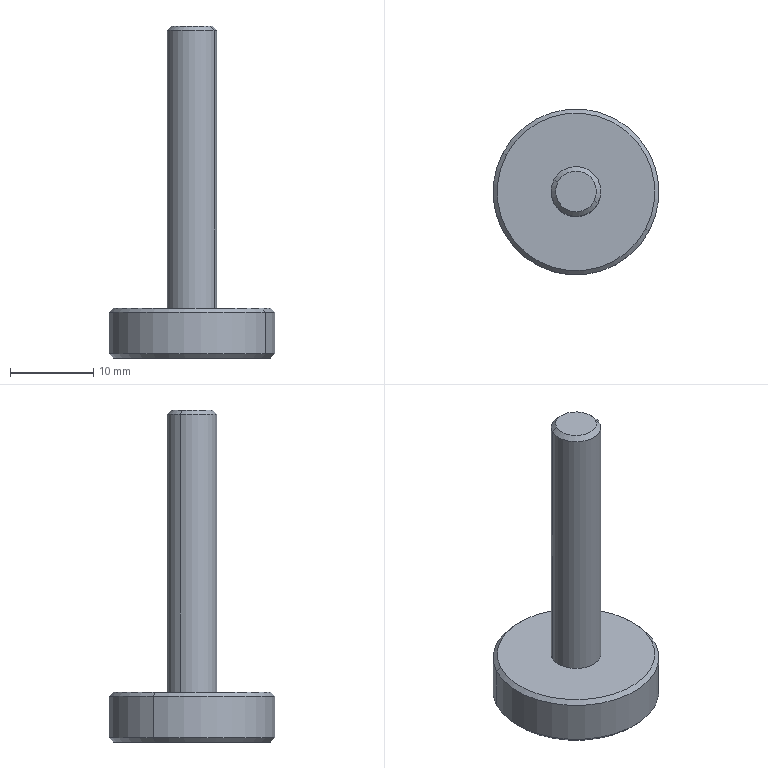Component | SolidWorks | 33KnurledScrew-1 | 1 solid | 13 faces | box 20 x 20 x 40 mm | volume 2828 mm3 | cone 6 | cylinder 4 | plane 3 | commonest cylinder face diameters 6 x2 20 x2
STEP:
#1=COLOUR_RGB('',0.7922,0.8196,0.9333);
#2=FILL_AREA_STYLE_COLOUR('',#1);
#3=FILL_AREA_STYLE('',(#2));
#4=SURFACE_STYLE_FILL_AREA(#3);
#5=SURFACE_SIDE_STYLE('',(#4));
#6=SURFACE_STYLE_USAGE(.BOTH.,#5);
#7=PRESENTATION_STYLE_ASSIGNMENT((#6));
#8=CARTESIAN_POINT('',(0.732,2.542,-5.276));
#9=VERTEX_POINT('',#8);
#10=CARTESIAN_POINT('',(0.07042,2.891,-5.276));
#11=VERTEX_POINT('',#10);
#12=CARTESIAN_POINT('',(0.4012,2.717,-5.276));
#13=DIRECTION('',(-0.,0.,1.));
#14=DIRECTION('',(0.8844,-0.4666,0.));
#15=AXIS2_PLACEMENT_3D('',#12,#13,#14);
#16=CIRCLE('',#15,0.374);
#17=EDGE_CURVE('',#9,#11,#16,.T.);
#18=ORIENTED_EDGE('',*,*,#17,.F.);
#19=CARTESIAN_POINT('',(0.7494,2.533,-5.295));
#20=VERTEX_POINT('',#19);
#21=CARTESIAN_POINT('',(0.732,2.542,-5.276));
#22=DIRECTION('',(0.6254,-0.33,-0.7071));
#23=VECTOR('',#22,39.37);
#24=LINE('',#21,#23);
#25=EDGE_CURVE('',#9,#20,#24,.T.);
#26=ORIENTED_EDGE('',*,*,#25,.T.);
#27=CARTESIAN_POINT('',(0.05301,2.9,-5.295));
#28=VERTEX_POINT('',#27);
#29=CARTESIAN_POINT('',(0.4012,2.717,-5.295));
#30=DIRECTION('',(0.,-0.,-1.));
#31=DIRECTION('',(0.8844,-0.4666,0.));
#32=AXIS2_PLACEMENT_3D('',#29,#30,#31);
#33=CIRCLE('',#32,0.3937);
#34=EDGE_CURVE('',#28,#20,#33,.T.);
#35=ORIENTED_EDGE('',*,*,#34,.F.);
#36=CARTESIAN_POINT('',(0.07042,2.891,-5.276));
#37=DIRECTION('',(-0.6254,0.33,-0.7071));
#38=VECTOR('',#37,39.37);
#39=LINE('',#36,#38);
#40=EDGE_CURVE('',#11,#28,#39,.T.);
#41=ORIENTED_EDGE('',*,*,#40,.F.);
#42=EDGE_LOOP('',(#18,#26,#35,#41));
#43=FACE_OUTER_BOUND('',#42,.T.);
#44=CARTESIAN_POINT('',(0.4012,2.717,-5.276));
#45=DIRECTION('',(0.,-0.,-1.));
#46=DIRECTION('',(-0.8844,0.4666,0.));
#47=AXIS2_PLACEMENT_3D('',#44,#45,#46);
#48=CONICAL_SURFACE('',#47,0.374,0.7854);
#49=ADVANCED_FACE('',(#43),#48,.T.);
#50=CARTESIAN_POINT('',(0.07042,2.891,-5.512));
#51=VERTEX_POINT('',#50);
#52=CARTESIAN_POINT('',(0.732,2.542,-5.512));
#53=VERTEX_POINT('',#52);
#54=CARTESIAN_POINT('',(0.4012,2.717,-5.512));
#55=DIRECTION('',(0.,-0.,-1.));
#56=DIRECTION('',(0.8844,-0.4666,0.));
#57=AXIS2_PLACEMENT_3D('',#54,#55,#56);
#58=CIRCLE('',#57,0.374);
#59=EDGE_CURVE('',#51,#53,#58,.T.);
#60=ORIENTED_EDGE('',*,*,#59,.F.);
#61=CARTESIAN_POINT('',(0.05301,2.9,-5.492));
#62=VERTEX_POINT('',#61);
#63=CARTESIAN_POINT('',(0.05301,2.9,-5.492));
#64=DIRECTION('',(-0.6254,0.33,0.7071));
#65=VECTOR('',#64,39.37);
#66=LINE('',#63,#65);
#67=EDGE_CURVE('',#51,#62,#66,.T.);
#68=ORIENTED_EDGE('',*,*,#67,.T.);
#69=CARTESIAN_POINT('',(0.7494,2.533,-5.492));
#70=VERTEX_POINT('',#69);
#71=CARTESIAN_POINT('',(0.4012,2.717,-5.492));
#72=DIRECTION('',(-0.,0.,1.));
#73=DIRECTION('',(0.8844,-0.4666,0.));
#74=AXIS2_PLACEMENT_3D('',#71,#72,#73);
#75=CIRCLE('',#74,0.3937);
#76=EDGE_CURVE('',#70,#62,#75,.T.);
#77=ORIENTED_EDGE('',*,*,#76,.F.);
#78=CARTESIAN_POINT('',(0.7494,2.533,-5.492));
#79=DIRECTION('',(0.6254,-0.33,0.7071));
#80=VECTOR('',#79,39.37);
#81=LINE('',#78,#80);
#82=EDGE_CURVE('',#53,#70,#81,.T.);
#83=ORIENTED_EDGE('',*,*,#82,.F.);
#84=EDGE_LOOP('',(#60,#68,#77,#83));
#85=FACE_OUTER_BOUND('',#84,.T.);
#86=CARTESIAN_POINT('',(0.4012,2.717,-5.492));
#87=DIRECTION('',(-0.,0.,1.));
#88=DIRECTION('',(0.8844,-0.4666,0.));
#89=AXIS2_PLACEMENT_3D('',#86,#87,#88);
#90=CONICAL_SURFACE('',#89,0.3937,0.7854);
#91=ADVANCED_FACE('',(#85),#90,.T.);
#92=CARTESIAN_POINT('',(0.3156,2.762,-3.937));
#93=VERTEX_POINT('',#92);
#94=CARTESIAN_POINT('',(0.4868,2.671,-3.937));
#95=VERTEX_POINT('',#94);
#96=CARTESIAN_POINT('',(0.4012,2.717,-3.937));
#97=DIRECTION('',(0.,-0.,-1.));
#98=DIRECTION('',(-0.8844,0.4666,0.));
#99=AXIS2_PLACEMENT_3D('',#96,#97,#98);
#100=CIRCLE('',#99,0.09679);
#101=EDGE_CURVE('',#93,#95,#100,.T.);
#102=ORIENTED_EDGE('',*,*,#101,.T.);
#103=CARTESIAN_POINT('',(0.5057,2.661,-3.958));
#104=VERTEX_POINT('',#103);
#105=CARTESIAN_POINT('',(0.4868,2.671,-3.937));
#106=DIRECTION('',(0.6254,-0.33,-0.7071));
#107=VECTOR('',#106,39.37);
#108=LINE('',#105,#107);
#109=EDGE_CURVE('',#95,#104,#108,.T.);
#110=ORIENTED_EDGE('',*,*,#109,.T.);
#111=CARTESIAN_POINT('',(0.2968,2.772,-3.958));
#112=VERTEX_POINT('',#111);
#113=CARTESIAN_POINT('',(0.4012,2.717,-3.958));
#114=DIRECTION('',(0.,-0.,-1.));
#115=DIRECTION('',(-0.8844,0.4666,0.));
#116=AXIS2_PLACEMENT_3D('',#113,#114,#115);
#117=CIRCLE('',#116,0.1181);
#118=EDGE_CURVE('',#112,#104,#117,.T.);
#119=ORIENTED_EDGE('',*,*,#118,.F.);
#120=CARTESIAN_POINT('',(0.3156,2.762,-3.937));
#121=DIRECTION('',(-0.6254,0.33,-0.7071));
#122=VECTOR('',#121,39.37);
#123=LINE('',#120,#122);
#124=EDGE_CURVE('',#93,#112,#123,.T.);
#125=ORIENTED_EDGE('',*,*,#124,.F.);
#126=EDGE_LOOP('',(#102,#110,#119,#125));
#127=FACE_OUTER_BOUND('',#126,.T.);
#128=CARTESIAN_POINT('',(0.4012,2.717,-3.937));
#129=DIRECTION('',(0.,-0.,-1.));
#130=DIRECTION('',(-0.8844,0.4666,0.));
#131=AXIS2_PLACEMENT_3D('',#128,#129,#130);
#132=CONICAL_SURFACE('',#131,0.09679,0.7854);
#133=ADVANCED_FACE('',(#127),#132,.T.);
#134=ORIENTED_EDGE('',*,*,#118,.T.);
#135=CARTESIAN_POINT('',(0.5057,2.661,-5.276));
#136=VERTEX_POINT('',#135);
#137=CARTESIAN_POINT('',(0.5057,2.661,-3.937));
#138=DIRECTION('',(0.,-0.,-1.));
#139=VECTOR('',#138,39.37);
#140=LINE('',#137,#139);
#141=EDGE_CURVE('',#104,#136,#140,.T.);
#142=ORIENTED_EDGE('',*,*,#141,.T.);
#143=CARTESIAN_POINT('',(0.2968,2.772,-5.276));
#144=VERTEX_POINT('',#143);
#145=CARTESIAN_POINT('',(0.4012,2.717,-5.276));
#146=DIRECTION('',(-0.,0.,1.));
#147=DIRECTION('',(0.8844,-0.4666,0.));
#148=AXIS2_PLACEMENT_3D('',#145,#146,#147);
#149=CIRCLE('',#148,0.1181);
#150=EDGE_CURVE('',#136,#144,#149,.T.);
#151=ORIENTED_EDGE('',*,*,#150,.T.);
#152=CARTESIAN_POINT('',(0.2968,2.772,-3.937));
#153=DIRECTION('',(0.,-0.,-1.));
#154=VECTOR('',#153,39.37);
#155=LINE('',#152,#154);
#156=EDGE_CURVE('',#112,#144,#155,.T.);
#157=ORIENTED_EDGE('',*,*,#156,.F.);
#158=EDGE_LOOP('',(#134,#142,#151,#157));
#159=FACE_OUTER_BOUND('',#158,.T.);
#160=CARTESIAN_POINT('',(0.4012,2.717,-3.937));
#161=DIRECTION('',(0.,-0.,-1.));
#162=DIRECTION('',(-0.8844,0.4666,0.));
#163=AXIS2_PLACEMENT_3D('',#160,#161,#162);
#164=CYLINDRICAL_SURFACE('',#163,0.1181);
#165=ADVANCED_FACE('',(#159),#164,.T.);
#166=ORIENTED_EDGE('',*,*,#34,.T.);
#167=CARTESIAN_POINT('',(0.7494,2.533,-5.276));
#168=DIRECTION('',(0.,-0.,-1.));
#169=VECTOR('',#168,39.37);
#170=LINE('',#167,#169);
#171=EDGE_CURVE('',#20,#70,#170,.T.);
#172=ORIENTED_EDGE('',*,*,#171,.T.);
#173=ORIENTED_EDGE('',*,*,#76,.T.);
#174=CARTESIAN_POINT('',(0.05301,2.9,-5.276));
#175=DIRECTION('',(0.,-0.,-1.));
#176=VECTOR('',#175,39.37);
#177=LINE('',#174,#176);
#178=EDGE_CURVE('',#28,#62,#177,.T.);
#179=ORIENTED_EDGE('',*,*,#178,.F.);
#180=EDGE_LOOP('',(#166,#172,#173,#179));
#181=FACE_OUTER_BOUND('',#180,.T.);
#182=CARTESIAN_POINT('',(0.4012,2.717,-5.276));
#183=DIRECTION('',(0.,-0.,-1.));
#184=DIRECTION('',(-0.8844,0.4666,0.));
#185=AXIS2_PLACEMENT_3D('',#182,#183,#184);
#186=CYLINDRICAL_SURFACE('',#185,0.3937);
#187=ADVANCED_FACE('',(#181),#186,.T.);
#188=ORIENTED_EDGE('',*,*,#171,.F.);
#189=CARTESIAN_POINT('',(0.4012,2.717,-5.295));
#190=DIRECTION('',(0.,-0.,-1.));
#191=DIRECTION('',(0.8844,-0.4666,0.));
#192=AXIS2_PLACEMENT_3D('',#189,#190,#191);
#193=CIRCLE('',#192,0.3937);
#194=EDGE_CURVE('',#20,#28,#193,.T.);
#195=ORIENTED_EDGE('',*,*,#194,.T.);
#196=ORIENTED_EDGE('',*,*,#178,.T.);
#197=CARTESIAN_POINT('',(0.4012,2.717,-5.492));
#198=DIRECTION('',(-0.,0.,1.));
#199=DIRECTION('',(0.8844,-0.4666,0.));
#200=AXIS2_PLACEMENT_3D('',#197,#198,#199);
#201=CIRCLE('',#200,0.3937);
#202=EDGE_CURVE('',#62,#70,#201,.T.);
#203=ORIENTED_EDGE('',*,*,#202,.T.);
#204=EDGE_LOOP('',(#188,#195,#196,#203));
#205=FACE_OUTER_BOUND('',#204,.T.);
#206=CARTESIAN_POINT('',(0.4012,2.717,-5.276));
#207=DIRECTION('',(0.,-0.,-1.));
#208=DIRECTION('',(-0.8844,0.4666,0.));
#209=AXIS2_PLACEMENT_3D('',#206,#207,#208);
#210=CYLINDRICAL_SURFACE('',#209,0.3937);
#211=ADVANCED_FACE('',(#205),#210,.T.);
#212=CARTESIAN_POINT('',(0.4012,2.717,-5.276));
#213=DIRECTION('',(-0.,0.,1.));
#214=DIRECTION('',(0.8844,-0.4666,0.));
#215=AXIS2_PLACEMENT_3D('',#212,#213,#214);
#216=CIRCLE('',#215,0.374);
#217=EDGE_CURVE('',#11,#9,#216,.T.);
#218=ORIENTED_EDGE('',*,*,#217,.T.);
#219=ORIENTED_EDGE('',*,*,#17,.T.);
#220=EDGE_LOOP('',(#218,#219));
#221=FACE_OUTER_BOUND('',#220,.T.);
#222=CARTESIAN_POINT('',(0.4012,2.717,-5.276));
#223=DIRECTION('',(-0.,0.,1.));
#224=DIRECTION('',(0.8844,-0.4666,0.));
#225=AXIS2_PLACEMENT_3D('',#222,#223,#224);
#226=CIRCLE('',#225,0.1181);
#227=EDGE_CURVE('',#144,#136,#226,.T.);
#228=ORIENTED_EDGE('',*,*,#227,.F.);
#229=ORIENTED_EDGE('',*,*,#150,.F.);
#230=EDGE_LOOP('',(#228,#229));
#231=FACE_BOUND('',#230,.T.);
#232=CARTESIAN_POINT('',(0.4012,2.717,-5.276));
#233=DIRECTION('',(-0.,0.,1.));
#234=DIRECTION('',(0.8844,-0.4666,0.));
#235=AXIS2_PLACEMENT_3D('',#232,#233,#234);
#236=PLANE('',#235);
#237=ADVANCED_FACE('',(#221,#231),#236,.T.);
#238=CARTESIAN_POINT('',(0.4012,2.717,-5.512));
#239=DIRECTION('',(0.,-0.,-1.));
#240=DIRECTION('',(0.8844,-0.4666,0.));
#241=AXIS2_PLACEMENT_3D('',#238,#239,#240);
#242=CIRCLE('',#241,0.374);
#243=EDGE_CURVE('',#53,#51,#242,.T.);
#244=ORIENTED_EDGE('',*,*,#243,.T.);
#245=ORIENTED_EDGE('',*,*,#59,.T.);
#246=EDGE_LOOP('',(#244,#245));
#247=FACE_OUTER_BOUND('',#246,.T.);
#248=CARTESIAN_POINT('',(0.4012,2.717,-5.512));
#249=DIRECTION('',(-0.,0.,1.));
#250=DIRECTION('',(0.8844,-0.4666,0.));
#251=AXIS2_PLACEMENT_3D('',#248,#249,#250);
#252=PLANE('',#251);
#253=ADVANCED_FACE('',(#247),#252,.F.);
#254=ORIENTED_EDGE('',*,*,#141,.F.);
#255=CARTESIAN_POINT('',(0.4012,2.717,-3.958));
#256=DIRECTION('',(0.,-0.,-1.));
#257=DIRECTION('',(-0.8844,0.4666,0.));
#258=AXIS2_PLACEMENT_3D('',#255,#256,#257);
#259=CIRCLE('',#258,0.1181);
#260=EDGE_CURVE('',#104,#112,#259,.T.);
#261=ORIENTED_EDGE('',*,*,#260,.T.);
#262=ORIENTED_EDGE('',*,*,#156,.T.);
#263=ORIENTED_EDGE('',*,*,#227,.T.);
#264=EDGE_LOOP('',(#254,#261,#262,#263));
#265=FACE_OUTER_BOUND('',#264,.T.);
#266=CARTESIAN_POINT('',(0.4012,2.717,-3.937));
#267=DIRECTION('',(0.,-0.,-1.));
#268=DIRECTION('',(-0.8844,0.4666,0.));
#269=AXIS2_PLACEMENT_3D('',#266,#267,#268);
#270=CYLINDRICAL_SURFACE('',#269,0.1181);
#271=ADVANCED_FACE('',(#265),#270,.T.);
#272=ORIENTED_EDGE('',*,*,#109,.F.);
#273=CARTESIAN_POINT('',(0.4012,2.717,-3.937));
#274=DIRECTION('',(0.,-0.,-1.));
#275=DIRECTION('',(-0.8844,0.4666,0.));
#276=AXIS2_PLACEMENT_3D('',#273,#274,#275);
#277=CIRCLE('',#276,0.09679);
#278=EDGE_CURVE('',#95,#93,#277,.T.);
#279=ORIENTED_EDGE('',*,*,#278,.T.);
#280=ORIENTED_EDGE('',*,*,#124,.T.);
#281=ORIENTED_EDGE('',*,*,#260,.F.);
#282=EDGE_LOOP('',(#272,#279,#280,#281));
#283=FACE_OUTER_BOUND('',#282,.T.);
#284=CARTESIAN_POINT('',(0.4012,2.717,-3.937));
#285=DIRECTION('',(0.,-0.,-1.));
#286=DIRECTION('',(-0.8844,0.4666,0.));
#287=AXIS2_PLACEMENT_3D('',#284,#285,#286);
#288=CONICAL_SURFACE('',#287,0.09679,0.7854);
#289=ADVANCED_FACE('',(#283),#288,.T.);
#290=ORIENTED_EDGE('',*,*,#101,.F.);
#291=ORIENTED_EDGE('',*,*,#278,.F.);
#292=EDGE_LOOP('',(#290,#291));
#293=FACE_OUTER_BOUND('',#292,.T.);
#294=CARTESIAN_POINT('',(0.4012,2.717,-3.937));
#295=DIRECTION('',(-0.,0.,1.));
#296=DIRECTION('',(0.8844,-0.4666,0.));
#297=AXIS2_PLACEMENT_3D('',#294,#295,#296);
#298=PLANE('',#297);
#299=ADVANCED_FACE('',(#293),#298,.T.);
#300=ORIENTED_EDGE('',*,*,#67,.F.);
#301=ORIENTED_EDGE('',*,*,#243,.F.);
#302=ORIENTED_EDGE('',*,*,#82,.T.);
#303=ORIENTED_EDGE('',*,*,#202,.F.);
#304=EDGE_LOOP('',(#300,#301,#302,#303));
#305=FACE_OUTER_BOUND('',#304,.T.);
#306=CARTESIAN_POINT('',(0.4012,2.717,-5.492));
#307=DIRECTION('',(-0.,0.,1.));
#308=DIRECTION('',(0.8844,-0.4666,0.));
#309=AXIS2_PLACEMENT_3D('',#306,#307,#308);
#310=CONICAL_SURFACE('',#309,0.3937,0.7854);
#311=ADVANCED_FACE('',(#305),#310,.T.);
#312=ORIENTED_EDGE('',*,*,#25,.F.);
#313=ORIENTED_EDGE('',*,*,#217,.F.);
#314=ORIENTED_EDGE('',*,*,#40,.T.);
#315=ORIENTED_EDGE('',*,*,#194,.F.);
#316=EDGE_LOOP('',(#312,#313,#314,#315));
#317=FACE_OUTER_BOUND('',#316,.T.);
#318=CARTESIAN_POINT('',(0.4012,2.717,-5.276));
#319=DIRECTION('',(0.,-0.,-1.));
#320=DIRECTION('',(-0.8844,0.4666,0.));
#321=AXIS2_PLACEMENT_3D('',#318,#319,#320);
#322=CONICAL_SURFACE('',#321,0.374,0.7854);
#323=ADVANCED_FACE('',(#317),#322,.T.);
#324=CLOSED_SHELL('',(#49,#91,#133,#165,#187,#211,#237,#253,#271,#289,#299,#311,#323));
#325=MANIFOLD_SOLID_BREP('',#324);
#326=STYLED_ITEM('',(#7),#325);
#327=(LENGTH_UNIT()NAMED_UNIT(*)SI_UNIT($,.METRE.));
#328=LENGTH_MEASURE_WITH_UNIT(LENGTH_MEASURE(0.0254),#327);
#329=DIMENSIONAL_EXPONENTS(1.,0.,0.,0.,0.,0.,0.);
#330=(CONVERSION_BASED_UNIT('',#328)LENGTH_UNIT()NAMED_UNIT(#329));
#331=UNCERTAINTY_MEASURE_WITH_UNIT(LENGTH_MEASURE(0.00001),#330,'','');
#332=(NAMED_UNIT(*)PLANE_ANGLE_UNIT()SI_UNIT($,.RADIAN.));
#333=(NAMED_UNIT(*)SI_UNIT($,.STERADIAN.)SOLID_ANGLE_UNIT());
#334=(GEOMETRIC_REPRESENTATION_CONTEXT(3)GLOBAL_UNCERTAINTY_ASSIGNED_CONTEXT((#331))GLOBAL_UNIT_ASSIGNED_CONTEXT((#330,#332,#333))REPRESENTATION_CONTEXT('',''));
#335=MECHANICAL_DESIGN_GEOMETRIC_PRESENTATION_REPRESENTATION('',(#326),#334);
#336=CARTESIAN_POINT('',(0.,0.,0.));
#337=DIRECTION('',(0.,0.,1.));
#338=DIRECTION('',(1.,0.,0.));
#339=AXIS2_PLACEMENT_3D('',#336,#337,#338);
#340=(LENGTH_UNIT()NAMED_UNIT(*)SI_UNIT($,.METRE.));
#341=LENGTH_MEASURE_WITH_UNIT(LENGTH_MEASURE(0.0254),#340);
#342=DIMENSIONAL_EXPONENTS(1.,0.,0.,0.,0.,0.,0.);
#343=(CONVERSION_BASED_UNIT('',#341)LENGTH_UNIT()NAMED_UNIT(#342));
#344=UNCERTAINTY_MEASURE_WITH_UNIT(LENGTH_MEASURE(0.00001),#343,'','');
#345=(NAMED_UNIT(*)PLANE_ANGLE_UNIT()SI_UNIT($,.RADIAN.));
#346=(NAMED_UNIT(*)SI_UNIT($,.STERADIAN.)SOLID_ANGLE_UNIT());
#347=(GEOMETRIC_REPRESENTATION_CONTEXT(3)GLOBAL_UNCERTAINTY_ASSIGNED_CONTEXT((#344))GLOBAL_UNIT_ASSIGNED_CONTEXT((#343,#345,#346))REPRESENTATION_CONTEXT('',''));
#348=ADVANCED_BREP_SHAPE_REPRESENTATION('',(#325,#339),#347);
#349=PRESENTATION_LAYER_ASSIGNMENT('','',(#326));